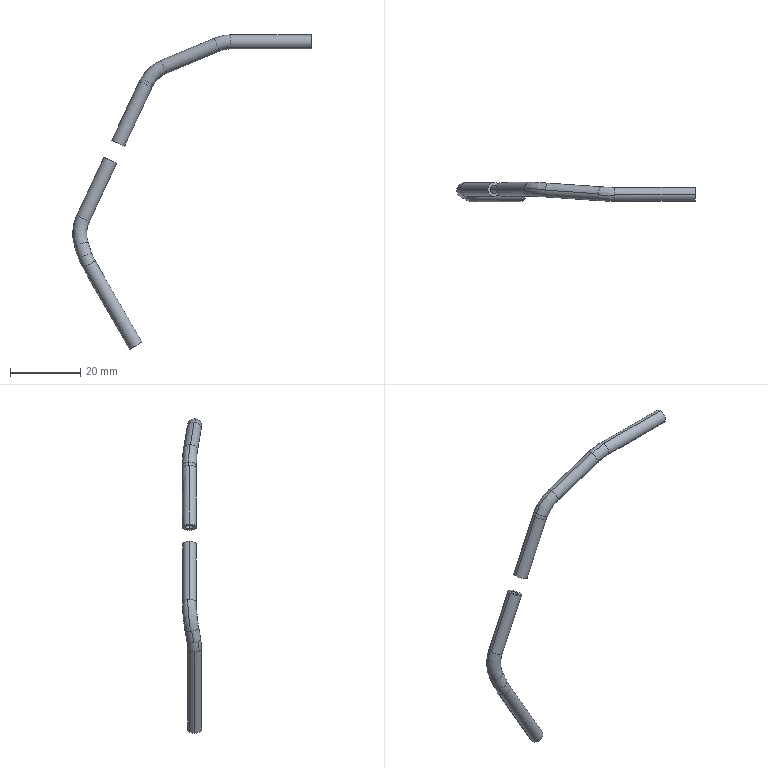Component | SolidWorks | WaterPipe3-1 | 2 solids | 48 faces | box 68.03 x 5.45 x 89.6 mm | volume 1031 mm3 | cylinder 24 | torus 20 | plane 4 | commonest cylinder face diameters 2.4 x12 4 x12
build123d program:
from build123d import *

# Parameters (mm, degrees)
SCAN_THIN_FEATURE1_PROFILE_R   = 2
SCAN_THIN_FEATURE1_PROFILE_R_2 = 1.2
CUT_EXTRUDE1_DEPTH             = 10


with BuildPart() as part:
    # Scan-Thin Feature1: sweep along a curve in space
    with BuildLine() as scan_thin_feature1_path:
        Line((-50, 0, -86.603), (-36.645, 0, -63.472))
        ThreePointArc((-35.159, 0.2103, -61.399), (-35.951, 0.05279, -62.395), (-36.645, 0, -63.472))
        Line((-35.159, 0.2103, -61.399), (-32.879, 0.7801, -58.811))
        ThreePointArc((-26.148, 1.446, -55.432), (-29.851, 1.273, -56.48), (-32.879, 0.7801, -58.811))
        Line((-26.148, 1.446, -55.432), (15.915, 1.446, -51.752))
        ThreePointArc((22.878, 1.194, -53.772), (19.588, 1.38, -52.111), (15.915, 1.446, -51.752))
        Line((22.878, 1.194, -53.772), (35.896, 0.131, -63.725))
        ThreePointArc((38.512, 0, -66.705), (37.351, 0.03308, -65.085), (35.896, 0.131, -63.725))
        Line((38.512, 0, -66.705), (50, 0, -86.603))
    # Scan-Thin Feature1 profile (on start of the path) → Scan-Thin Feature1 (sweep)
    with BuildSketch(Plane(origin=(-50, 0, -86.603), x_dir=(0.866, 0, -0.5), z_dir=(0.5, 0, 0.866))):
        Circle(SCAN_THIN_FEATURE1_PROFILE_R)
        Circle(SCAN_THIN_FEATURE1_PROFILE_R_2, mode=Mode.SUBTRACT)
    sweep(path=scan_thin_feature1_path.line)

    # Sketch6 → Cut-Extrude1 (cut, symmetric)
    with BuildSketch(Plane(origin=(0, 0, 0), x_dir=(1, 0, 0), z_dir=(0, 1, 0))):
        Polygon((-2.287, 56.054), (-7.666, 56.525), (-8.137, 51.146), (-2.757, 50.675), align=None)
    extrude(amount=CUT_EXTRUDE1_DEPTH, both=True, mode=Mode.SUBTRACT)


with BuildPart() as cut_extrude1_piece_1:
    # of the separate pieces the step leaves, piece 1, a body of its own (cut_extrude1_pieces)
    add(part.part.solids().sort_by_distance((-2.348, 1.282, -55.35))[0])


with BuildPart() as cut_extrude1_piece_2:
    # of the separate pieces the step leaves, piece 2, a body of its own (cut_extrude1_pieces)
    add(part.part.solids().sort_by_distance((-48.268, 0, -87.603))[0])


solid = Compound([cut_extrude1_piece_1.part, cut_extrude1_piece_2.part])

# Placed as in the assembly
solid = solid.moved(Location((-116.947, 33.561, 224.066), (0, -60, 0)))